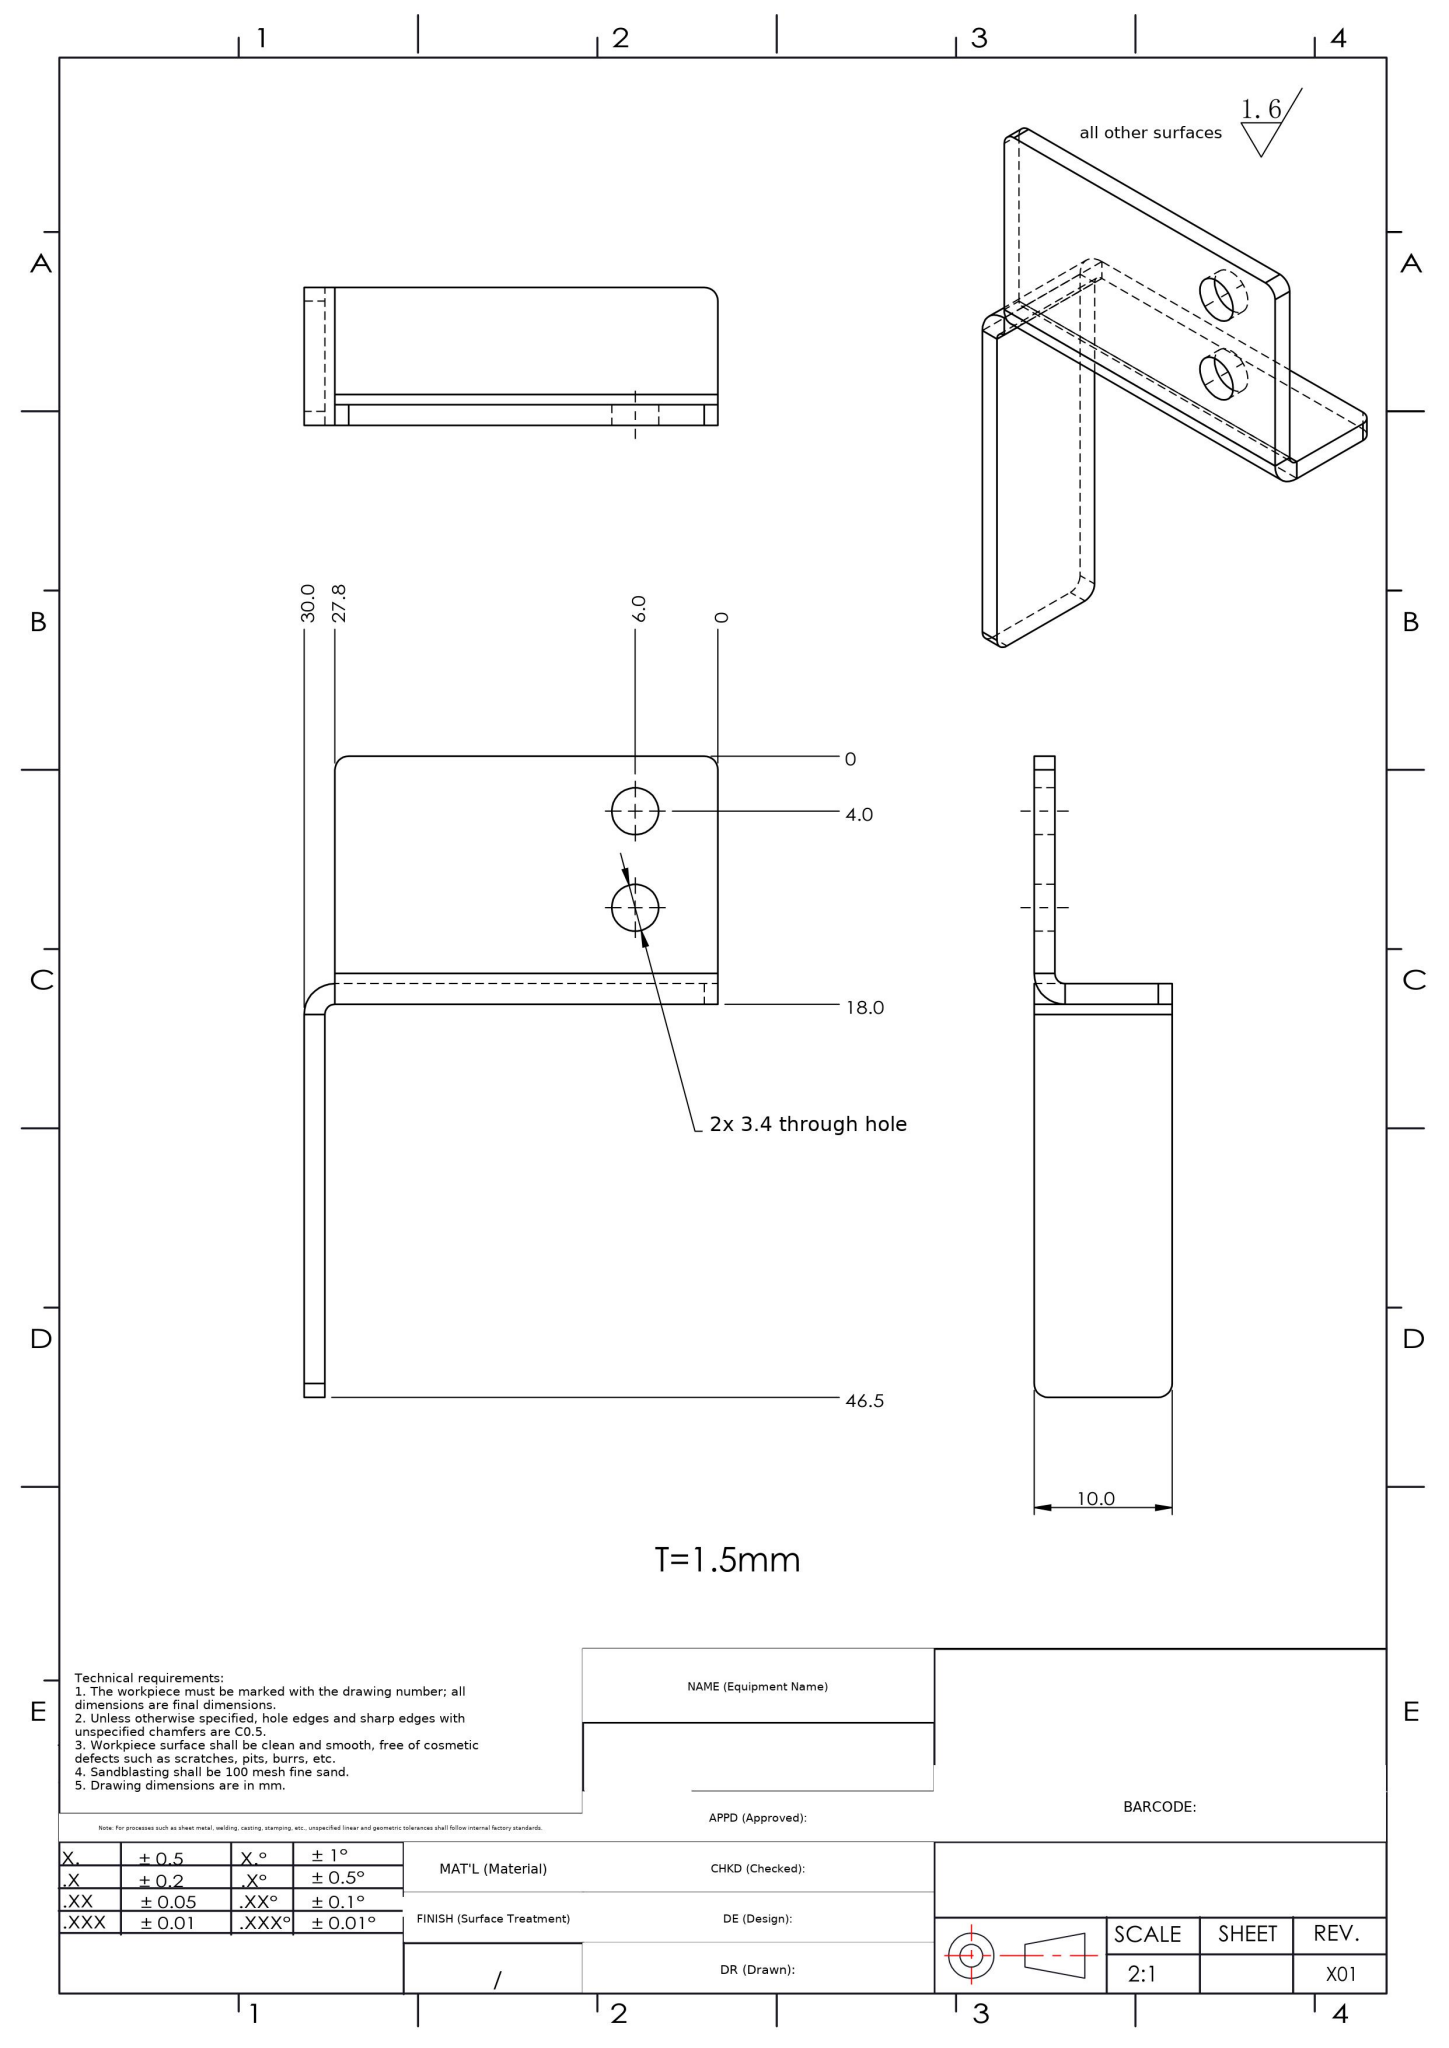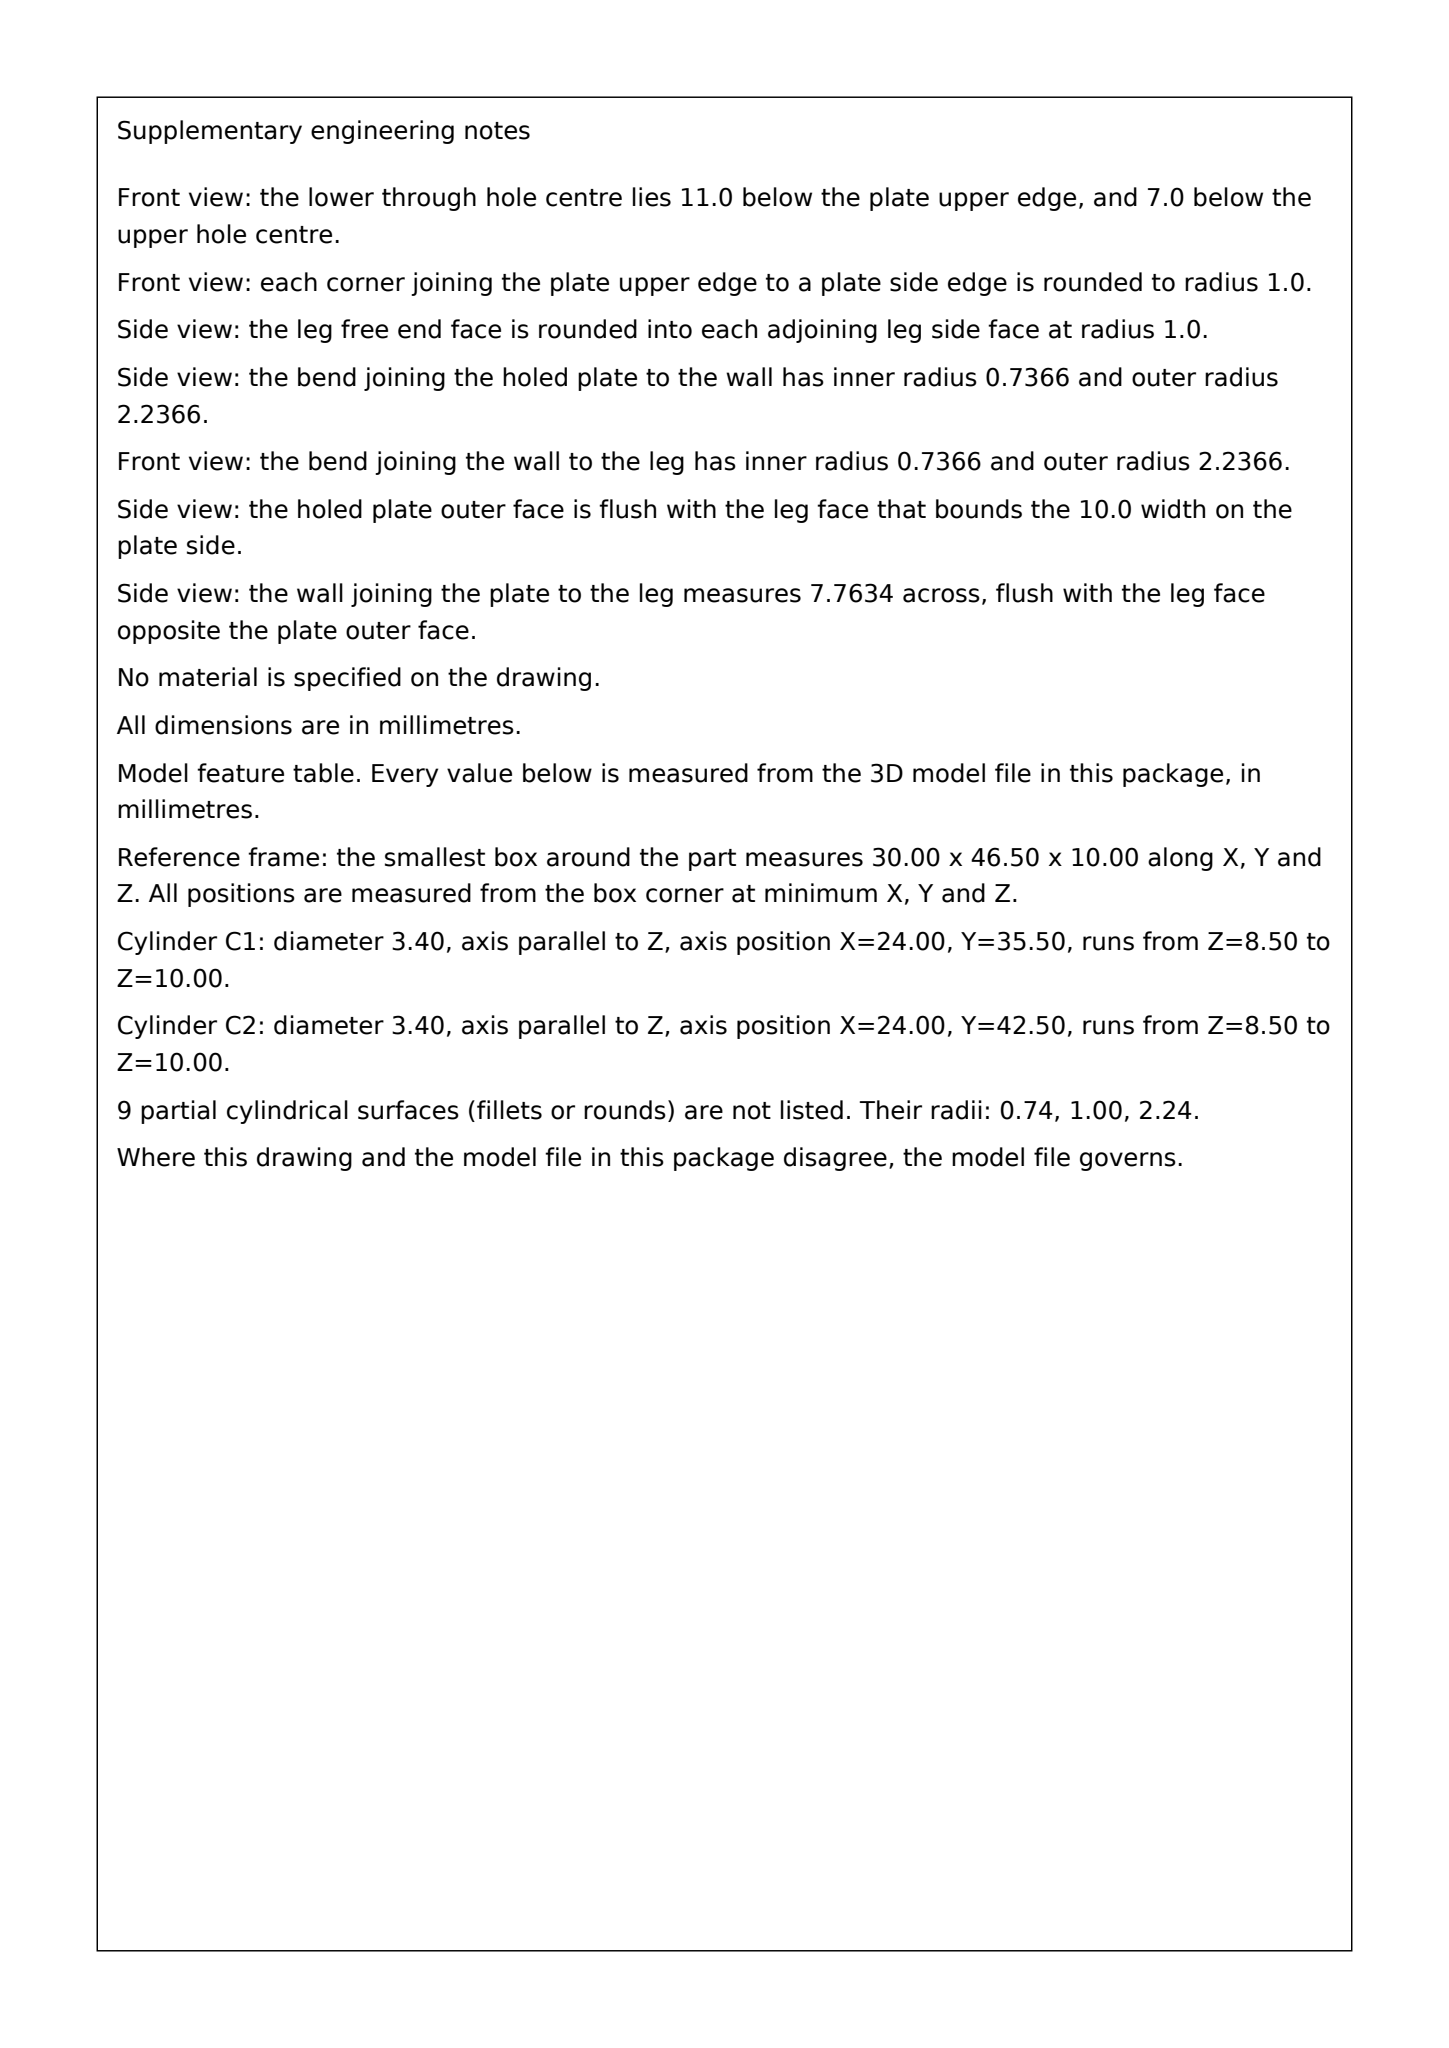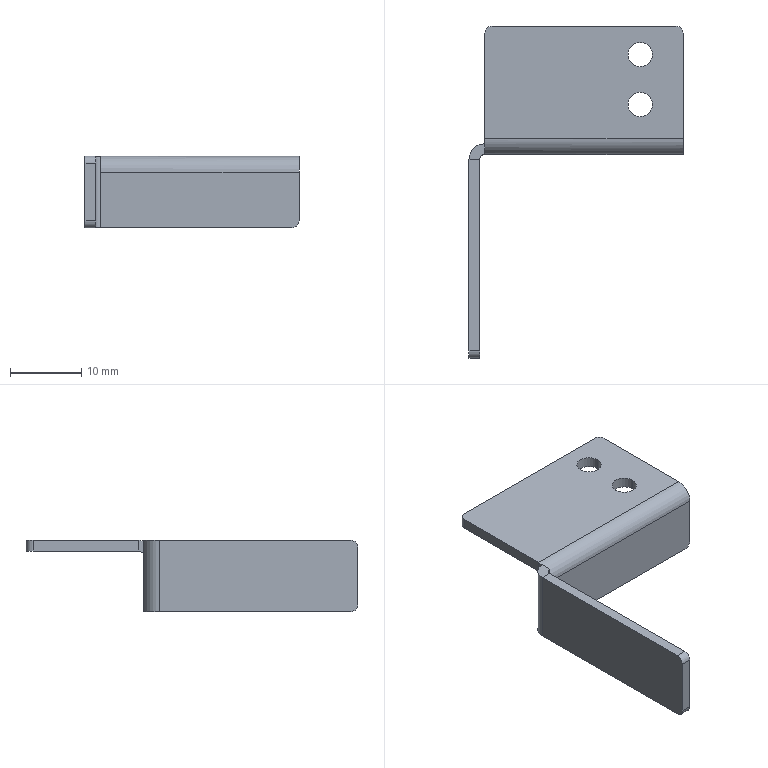Part | SolidWorks | mm | 1 solid | 32 faces | box 30 x 46.5 x 10 mm | volume 1500 mm3 | plane 19 | cylinder 13 | commonest cylinder face diameters 2 x5 3.4 x4 4.473 x2 1.473 x2
Drawing notes:
2X 90° BEND: INSIDE R0.74, OUTSIDE R2.24, T=1.5 | from the solid: Bend cylinders dia 1.473 (R0.736 inner) & dia 4.473 (R2.236 outer), axes x@[30.74,7.76] L27.76 and z@[2.24,27.76] L10.0; thickness 1.5
STEP:
#1=CARTESIAN_POINT('',(25.7,42.5,10.));
#2=VERTEX_POINT('',#1);
#3=CARTESIAN_POINT('',(22.3,42.5,10.));
#4=VERTEX_POINT('',#3);
#5=CARTESIAN_POINT('',(24.,42.5,10.));
#6=DIRECTION('',(0.,0.,-1.));
#7=DIRECTION('',(-1.,0.,0.));
#8=AXIS2_PLACEMENT_3D('',#5,#6,#7);
#9=CIRCLE('',#8,1.7);
#10=EDGE_CURVE('',#2,#4,#9,.T.);
#11=ORIENTED_EDGE('',*,*,#10,.F.);
#12=CARTESIAN_POINT('',(25.7,42.5,8.5));
#13=VERTEX_POINT('',#12);
#14=CARTESIAN_POINT('',(25.7,42.5,8.5));
#15=DIRECTION('',(0.,0.,-1.));
#16=VECTOR('',#15,1000.);
#17=LINE('',#14,#16);
#18=EDGE_CURVE('',#2,#13,#17,.T.);
#19=ORIENTED_EDGE('',*,*,#18,.T.);
#20=CARTESIAN_POINT('',(22.3,42.5,8.5));
#21=VERTEX_POINT('',#20);
#22=CARTESIAN_POINT('',(24.,42.5,8.5));
#23=DIRECTION('',(0.,0.,-1.));
#24=DIRECTION('',(-1.,0.,0.));
#25=AXIS2_PLACEMENT_3D('',#22,#23,#24);
#26=CIRCLE('',#25,1.7);
#27=EDGE_CURVE('',#13,#21,#26,.T.);
#28=ORIENTED_EDGE('',*,*,#27,.T.);
#29=CARTESIAN_POINT('',(22.3,42.5,8.5));
#30=DIRECTION('',(0.,0.,-1.));
#31=VECTOR('',#30,1000.);
#32=LINE('',#29,#31);
#33=EDGE_CURVE('',#4,#21,#32,.T.);
#34=ORIENTED_EDGE('',*,*,#33,.F.);
#35=EDGE_LOOP('',(#11,#19,#28,#34));
#36=FACE_OUTER_BOUND('',#35,.T.);
#37=CARTESIAN_POINT('',(24.,42.5,8.5));
#38=DIRECTION('',(0.,0.,-1.));
#39=DIRECTION('',(-1.,0.,0.));
#40=AXIS2_PLACEMENT_3D('',#37,#38,#39);
#41=CYLINDRICAL_SURFACE('',#40,1.7);
#42=ADVANCED_FACE('',(#36),#41,.F.);
#43=CARTESIAN_POINT('',(25.7,35.5,10.));
#44=VERTEX_POINT('',#43);
#45=CARTESIAN_POINT('',(22.3,35.5,10.));
#46=VERTEX_POINT('',#45);
#47=CARTESIAN_POINT('',(24.,35.5,10.));
#48=DIRECTION('',(0.,0.,-1.));
#49=DIRECTION('',(-1.,0.,0.));
#50=AXIS2_PLACEMENT_3D('',#47,#48,#49);
#51=CIRCLE('',#50,1.7);
#52=EDGE_CURVE('',#44,#46,#51,.T.);
#53=ORIENTED_EDGE('',*,*,#52,.F.);
#54=CARTESIAN_POINT('',(25.7,35.5,8.5));
#55=VERTEX_POINT('',#54);
#56=CARTESIAN_POINT('',(25.7,35.5,8.5));
#57=DIRECTION('',(0.,0.,-1.));
#58=VECTOR('',#57,1000.);
#59=LINE('',#56,#58);
#60=EDGE_CURVE('',#44,#55,#59,.T.);
#61=ORIENTED_EDGE('',*,*,#60,.T.);
#62=CARTESIAN_POINT('',(22.3,35.5,8.5));
#63=VERTEX_POINT('',#62);
#64=CARTESIAN_POINT('',(24.,35.5,8.5));
#65=DIRECTION('',(0.,0.,-1.));
#66=DIRECTION('',(-1.,0.,0.));
#67=AXIS2_PLACEMENT_3D('',#64,#65,#66);
#68=CIRCLE('',#67,1.7);
#69=EDGE_CURVE('',#55,#63,#68,.T.);
#70=ORIENTED_EDGE('',*,*,#69,.T.);
#71=CARTESIAN_POINT('',(22.3,35.5,8.5));
#72=DIRECTION('',(0.,0.,-1.));
#73=VECTOR('',#72,1000.);
#74=LINE('',#71,#73);
#75=EDGE_CURVE('',#46,#63,#74,.T.);
#76=ORIENTED_EDGE('',*,*,#75,.F.);
#77=EDGE_LOOP('',(#53,#61,#70,#76));
#78=FACE_OUTER_BOUND('',#77,.T.);
#79=CARTESIAN_POINT('',(24.,35.5,8.5));
#80=DIRECTION('',(0.,0.,-1.));
#81=DIRECTION('',(-1.,0.,0.));
#82=AXIS2_PLACEMENT_3D('',#79,#80,#81);
#83=CYLINDRICAL_SURFACE('',#82,1.7);
#84=ADVANCED_FACE('',(#78),#83,.F.);
#85=CARTESIAN_POINT('',(2.237,28.5,10.));
#86=VERTEX_POINT('',#85);
#87=CARTESIAN_POINT('',(2.237,28.5,7.763));
#88=VERTEX_POINT('',#87);
#89=CARTESIAN_POINT('',(2.237,28.5,10.));
#90=DIRECTION('',(0.,0.,-1.));
#91=VECTOR('',#90,1000.);
#92=LINE('',#89,#91);
#93=EDGE_CURVE('',#86,#88,#92,.T.);
#94=ORIENTED_EDGE('',*,*,#93,.T.);
#95=CARTESIAN_POINT('',(2.237,30.,9.875));
#96=VERTEX_POINT('',#95);
#97=CARTESIAN_POINT('',(2.237,30.737,7.763));
#98=DIRECTION('',(-1.,0.,0.));
#99=DIRECTION('',(0.,0.,-1.));
#100=AXIS2_PLACEMENT_3D('',#97,#98,#99);
#101=CIRCLE('',#100,2.237);
#102=EDGE_CURVE('',#88,#96,#101,.T.);
#103=ORIENTED_EDGE('',*,*,#102,.T.);
#104=CARTESIAN_POINT('',(2.237,30.,10.));
#105=VERTEX_POINT('',#104);
#106=CARTESIAN_POINT('',(2.237,30.,10.));
#107=DIRECTION('',(0.,0.,-1.));
#108=VECTOR('',#107,1000.);
#109=LINE('',#106,#108);
#110=EDGE_CURVE('',#105,#96,#109,.T.);
#111=ORIENTED_EDGE('',*,*,#110,.F.);
#112=CARTESIAN_POINT('',(2.237,30.,10.));
#113=DIRECTION('',(0.,-1.,0.));
#114=VECTOR('',#113,1000.);
#115=LINE('',#112,#114);
#116=EDGE_CURVE('',#105,#86,#115,.T.);
#117=ORIENTED_EDGE('',*,*,#116,.T.);
#118=EDGE_LOOP('',(#94,#103,#111,#117));
#119=FACE_OUTER_BOUND('',#118,.T.);
#120=CARTESIAN_POINT('',(2.237,30.,7.763));
#121=DIRECTION('',(1.,0.,0.));
#122=DIRECTION('',(0.,0.,-1.));
#123=AXIS2_PLACEMENT_3D('',#120,#121,#122);
#124=PLANE('',#123);
#125=ADVANCED_FACE('',(#119),#124,.T.);
#126=CARTESIAN_POINT('',(2.237,28.5,0.));
#127=VERTEX_POINT('',#126);
#128=CARTESIAN_POINT('',(29.,28.5,0.));
#129=VERTEX_POINT('',#128);
#130=CARTESIAN_POINT('',(0.,28.5,0.));
#131=DIRECTION('',(1.,0.,0.));
#132=VECTOR('',#131,1000.);
#133=LINE('',#130,#132);
#134=EDGE_CURVE('',#127,#129,#133,.T.);
#135=ORIENTED_EDGE('',*,*,#134,.T.);
#136=CARTESIAN_POINT('',(30.,28.5,1.));
#137=VERTEX_POINT('',#136);
#138=CARTESIAN_POINT('',(29.,28.5,1.));
#139=DIRECTION('',(0.,-1.,0.));
#140=DIRECTION('',(0.,0.,1.));
#141=AXIS2_PLACEMENT_3D('',#138,#139,#140);
#142=CIRCLE('',#141,1.);
#143=EDGE_CURVE('',#129,#137,#142,.T.);
#144=ORIENTED_EDGE('',*,*,#143,.T.);
#145=CARTESIAN_POINT('',(30.,28.5,7.763));
#146=VERTEX_POINT('',#145);
#147=CARTESIAN_POINT('',(30.,28.5,10.));
#148=DIRECTION('',(0.,0.,-1.));
#149=VECTOR('',#148,1000.);
#150=LINE('',#147,#149);
#151=EDGE_CURVE('',#146,#137,#150,.T.);
#152=ORIENTED_EDGE('',*,*,#151,.F.);
#153=CARTESIAN_POINT('',(30.,28.5,7.763));
#154=DIRECTION('',(-1.,0.,0.));
#155=VECTOR('',#154,1000.);
#156=LINE('',#153,#155);
#157=EDGE_CURVE('',#146,#88,#156,.T.);
#158=ORIENTED_EDGE('',*,*,#157,.T.);
#159=CARTESIAN_POINT('',(2.237,28.5,10.));
#160=DIRECTION('',(0.,0.,-1.));
#161=VECTOR('',#160,1000.);
#162=LINE('',#159,#161);
#163=EDGE_CURVE('',#88,#127,#162,.T.);
#164=ORIENTED_EDGE('',*,*,#163,.T.);
#165=EDGE_LOOP('',(#135,#144,#152,#158,#164));
#166=FACE_OUTER_BOUND('',#165,.T.);
#167=CARTESIAN_POINT('',(0.,28.5,10.));
#168=DIRECTION('',(0.,1.,0.));
#169=DIRECTION('',(0.,0.,1.));
#170=AXIS2_PLACEMENT_3D('',#167,#168,#169);
#171=PLANE('',#170);
#172=ADVANCED_FACE('',(#166),#171,.F.);
#173=ORIENTED_EDGE('',*,*,#151,.T.);
#174=CARTESIAN_POINT('',(30.,30.,1.));
#175=VERTEX_POINT('',#174);
#176=CARTESIAN_POINT('',(30.,30.,1.));
#177=DIRECTION('',(0.,1.,0.));
#178=VECTOR('',#177,1000.);
#179=LINE('',#176,#178);
#180=EDGE_CURVE('',#137,#175,#179,.T.);
#181=ORIENTED_EDGE('',*,*,#180,.T.);
#182=CARTESIAN_POINT('',(30.,30.,7.763));
#183=VERTEX_POINT('',#182);
#184=CARTESIAN_POINT('',(30.,30.,10.));
#185=DIRECTION('',(0.,0.,-1.));
#186=VECTOR('',#185,1000.);
#187=LINE('',#184,#186);
#188=EDGE_CURVE('',#183,#175,#187,.T.);
#189=ORIENTED_EDGE('',*,*,#188,.F.);
#190=CARTESIAN_POINT('',(30.,30.,7.763));
#191=DIRECTION('',(0.,-1.,0.));
#192=VECTOR('',#191,1000.);
#193=LINE('',#190,#192);
#194=EDGE_CURVE('',#183,#146,#193,.T.);
#195=ORIENTED_EDGE('',*,*,#194,.T.);
#196=EDGE_LOOP('',(#173,#181,#189,#195));
#197=FACE_OUTER_BOUND('',#196,.T.);
#198=CARTESIAN_POINT('',(30.,30.,10.));
#199=DIRECTION('',(1.,0.,0.));
#200=DIRECTION('',(0.,0.,-1.));
#201=AXIS2_PLACEMENT_3D('',#198,#199,#200);
#202=PLANE('',#201);
#203=ADVANCED_FACE('',(#197),#202,.T.);
#204=ORIENTED_EDGE('',*,*,#188,.T.);
#205=CARTESIAN_POINT('',(29.,30.,0.));
#206=VERTEX_POINT('',#205);
#207=CARTESIAN_POINT('',(29.,30.,1.));
#208=DIRECTION('',(0.,1.,0.));
#209=DIRECTION('',(0.,0.,1.));
#210=AXIS2_PLACEMENT_3D('',#207,#208,#209);
#211=CIRCLE('',#210,1.);
#212=EDGE_CURVE('',#175,#206,#211,.T.);
#213=ORIENTED_EDGE('',*,*,#212,.T.);
#214=CARTESIAN_POINT('',(2.237,30.,0.));
#215=VERTEX_POINT('',#214);
#216=CARTESIAN_POINT('',(0.,30.,0.));
#217=DIRECTION('',(1.,0.,0.));
#218=VECTOR('',#217,1000.);
#219=LINE('',#216,#218);
#220=EDGE_CURVE('',#215,#206,#219,.T.);
#221=ORIENTED_EDGE('',*,*,#220,.F.);
#222=CARTESIAN_POINT('',(2.237,30.,7.763));
#223=VERTEX_POINT('',#222);
#224=CARTESIAN_POINT('',(2.237,30.,10.));
#225=DIRECTION('',(0.,0.,-1.));
#226=VECTOR('',#225,1000.);
#227=LINE('',#224,#226);
#228=EDGE_CURVE('',#223,#215,#227,.T.);
#229=ORIENTED_EDGE('',*,*,#228,.F.);
#230=CARTESIAN_POINT('',(30.,30.,7.763));
#231=DIRECTION('',(-1.,0.,0.));
#232=VECTOR('',#231,1000.);
#233=LINE('',#230,#232);
#234=EDGE_CURVE('',#183,#223,#233,.T.);
#235=ORIENTED_EDGE('',*,*,#234,.F.);
#236=EDGE_LOOP('',(#204,#213,#221,#229,#235));
#237=FACE_OUTER_BOUND('',#236,.T.);
#238=CARTESIAN_POINT('',(0.,30.,10.));
#239=DIRECTION('',(0.,1.,0.));
#240=DIRECTION('',(0.,0.,1.));
#241=AXIS2_PLACEMENT_3D('',#238,#239,#240);
#242=PLANE('',#241);
#243=ADVANCED_FACE('',(#237),#242,.T.);
#244=ORIENTED_EDGE('',*,*,#116,.F.);
#245=CARTESIAN_POINT('',(0.,27.763,10.));
#246=VERTEX_POINT('',#245);
#247=CARTESIAN_POINT('',(2.237,27.763,10.));
#248=DIRECTION('',(0.,0.,-1.));
#249=DIRECTION('',(1.,0.,0.));
#250=AXIS2_PLACEMENT_3D('',#247,#248,#249);
#251=CIRCLE('',#250,2.237);
#252=EDGE_CURVE('',#246,#105,#251,.T.);
#253=ORIENTED_EDGE('',*,*,#252,.F.);
#254=CARTESIAN_POINT('',(1.5,27.763,10.));
#255=VERTEX_POINT('',#254);
#256=CARTESIAN_POINT('',(1.5,27.763,10.));
#257=DIRECTION('',(-1.,0.,0.));
#258=VECTOR('',#257,1000.);
#259=LINE('',#256,#258);
#260=EDGE_CURVE('',#255,#246,#259,.T.);
#261=ORIENTED_EDGE('',*,*,#260,.F.);
#262=CARTESIAN_POINT('',(2.237,27.763,10.));
#263=DIRECTION('',(0.,0.,-1.));
#264=DIRECTION('',(1.,0.,0.));
#265=AXIS2_PLACEMENT_3D('',#262,#263,#264);
#266=CIRCLE('',#265,0.7366);
#267=EDGE_CURVE('',#255,#86,#266,.T.);
#268=ORIENTED_EDGE('',*,*,#267,.T.);
#269=EDGE_LOOP('',(#244,#253,#261,#268));
#270=FACE_OUTER_BOUND('',#269,.T.);
#271=CARTESIAN_POINT('',(2.237,30.,10.));
#272=DIRECTION('',(0.,0.,1.));
#273=DIRECTION('',(1.,0.,0.));
#274=AXIS2_PLACEMENT_3D('',#271,#272,#273);
#275=PLANE('',#274);
#276=ADVANCED_FACE('',(#270),#275,.T.);
#277=CARTESIAN_POINT('',(0.,27.763,0.));
#278=VERTEX_POINT('',#277);
#279=CARTESIAN_POINT('',(1.5,27.763,0.));
#280=VERTEX_POINT('',#279);
#281=CARTESIAN_POINT('',(0.,27.763,0.));
#282=DIRECTION('',(1.,0.,0.));
#283=VECTOR('',#282,1000.);
#284=LINE('',#281,#283);
#285=EDGE_CURVE('',#278,#280,#284,.T.);
#286=ORIENTED_EDGE('',*,*,#285,.F.);
#287=CARTESIAN_POINT('',(2.237,27.763,0.));
#288=DIRECTION('',(0.,0.,-1.));
#289=DIRECTION('',(1.,0.,0.));
#290=AXIS2_PLACEMENT_3D('',#287,#288,#289);
#291=CIRCLE('',#290,2.237);
#292=EDGE_CURVE('',#278,#215,#291,.T.);
#293=ORIENTED_EDGE('',*,*,#292,.T.);
#294=CARTESIAN_POINT('',(2.237,28.5,0.));
#295=DIRECTION('',(0.,1.,0.));
#296=VECTOR('',#295,1000.);
#297=LINE('',#294,#296);
#298=EDGE_CURVE('',#127,#215,#297,.T.);
#299=ORIENTED_EDGE('',*,*,#298,.F.);
#300=CARTESIAN_POINT('',(2.237,27.763,0.));
#301=DIRECTION('',(0.,0.,-1.));
#302=DIRECTION('',(1.,0.,0.));
#303=AXIS2_PLACEMENT_3D('',#300,#301,#302);
#304=CIRCLE('',#303,0.7366);
#305=EDGE_CURVE('',#280,#127,#304,.T.);
#306=ORIENTED_EDGE('',*,*,#305,.F.);
#307=EDGE_LOOP('',(#286,#293,#299,#306));
#308=FACE_OUTER_BOUND('',#307,.T.);
#309=CARTESIAN_POINT('',(0.,27.763,0.));
#310=DIRECTION('',(0.,0.,-1.));
#311=DIRECTION('',(-1.,0.,0.));
#312=AXIS2_PLACEMENT_3D('',#309,#310,#311);
#313=PLANE('',#312);
#314=ADVANCED_FACE('',(#308),#313,.T.);
#315=CARTESIAN_POINT('',(1.5,1.,0.));
#316=VERTEX_POINT('',#315);
#317=CARTESIAN_POINT('',(1.5,0.,0.));
#318=DIRECTION('',(0.,1.,0.));
#319=VECTOR('',#318,1000.);
#320=LINE('',#317,#319);
#321=EDGE_CURVE('',#316,#280,#320,.T.);
#322=ORIENTED_EDGE('',*,*,#321,.F.);
#323=CARTESIAN_POINT('',(0.,1.,0.));
#324=VERTEX_POINT('',#323);
#325=CARTESIAN_POINT('',(2.237,1.,0.));
#326=DIRECTION('',(-1.,0.,0.));
#327=VECTOR('',#326,1000.);
#328=LINE('',#325,#327);
#329=EDGE_CURVE('',#316,#324,#328,.T.);
#330=ORIENTED_EDGE('',*,*,#329,.T.);
#331=CARTESIAN_POINT('',(0.,0.,0.));
#332=DIRECTION('',(0.,1.,0.));
#333=VECTOR('',#332,1000.);
#334=LINE('',#331,#333);
#335=EDGE_CURVE('',#324,#278,#334,.T.);
#336=ORIENTED_EDGE('',*,*,#335,.T.);
#337=ORIENTED_EDGE('',*,*,#285,.T.);
#338=EDGE_LOOP('',(#322,#330,#336,#337));
#339=FACE_OUTER_BOUND('',#338,.T.);
#340=CARTESIAN_POINT('',(2.237,28.5,0.));
#341=DIRECTION('',(0.,0.,-1.));
#342=DIRECTION('',(-1.,0.,0.));
#343=AXIS2_PLACEMENT_3D('',#340,#341,#342);
#344=PLANE('',#343);
#345=ADVANCED_FACE('',(#339),#344,.T.);
#346=ORIENTED_EDGE('',*,*,#292,.F.);
#347=CARTESIAN_POINT('',(0.,27.763,10.));
#348=DIRECTION('',(0.,0.,-1.));
#349=VECTOR('',#348,1000.);
#350=LINE('',#347,#349);
#351=EDGE_CURVE('',#246,#278,#350,.T.);
#352=ORIENTED_EDGE('',*,*,#351,.F.);
#353=ORIENTED_EDGE('',*,*,#252,.T.);
#354=ORIENTED_EDGE('',*,*,#110,.T.);
#355=CARTESIAN_POINT('',(2.237,30.,10.));
#356=DIRECTION('',(0.,0.,-1.));
#357=VECTOR('',#356,1000.);
#358=LINE('',#355,#357);
#359=EDGE_CURVE('',#96,#223,#358,.T.);
#360=ORIENTED_EDGE('',*,*,#359,.T.);
#361=ORIENTED_EDGE('',*,*,#228,.T.);
#362=EDGE_LOOP('',(#346,#352,#353,#354,#360,#361));
#363=FACE_OUTER_BOUND('',#362,.T.);
#364=CARTESIAN_POINT('',(2.237,27.763,10.));
#365=DIRECTION('',(0.,0.,-1.));
#366=DIRECTION('',(-1.,0.,0.));
#367=AXIS2_PLACEMENT_3D('',#364,#365,#366);
#368=CYLINDRICAL_SURFACE('',#367,2.237);
#369=ADVANCED_FACE('',(#363),#368,.T.);
#370=ORIENTED_EDGE('',*,*,#335,.F.);
#371=CARTESIAN_POINT('',(0.,0.,1.));
#372=VERTEX_POINT('',#371);
#373=CARTESIAN_POINT('',(0.,1.,1.));
#374=DIRECTION('',(-1.,0.,0.));
#375=DIRECTION('',(0.,0.,1.));
#376=AXIS2_PLACEMENT_3D('',#373,#374,#375);
#377=CIRCLE('',#376,1.);
#378=EDGE_CURVE('',#324,#372,#377,.T.);
#379=ORIENTED_EDGE('',*,*,#378,.T.);
#380=CARTESIAN_POINT('',(0.,0.,9.));
#381=VERTEX_POINT('',#380);
#382=CARTESIAN_POINT('',(0.,0.,10.));
#383=DIRECTION('',(0.,0.,-1.));
#384=VECTOR('',#383,1000.);
#385=LINE('',#382,#384);
#386=EDGE_CURVE('',#381,#372,#385,.T.);
#387=ORIENTED_EDGE('',*,*,#386,.F.);
#388=CARTESIAN_POINT('',(0.,1.,10.));
#389=VERTEX_POINT('',#388);
#390=CARTESIAN_POINT('',(0.,1.,9.));
#391=DIRECTION('',(-1.,0.,0.));
#392=DIRECTION('',(0.,0.,1.));
#393=AXIS2_PLACEMENT_3D('',#390,#391,#392);
#394=CIRCLE('',#393,1.);
#395=EDGE_CURVE('',#381,#389,#394,.T.);
#396=ORIENTED_EDGE('',*,*,#395,.T.);
#397=CARTESIAN_POINT('',(0.,0.,10.));
#398=DIRECTION('',(0.,1.,0.));
#399=VECTOR('',#398,1000.);
#400=LINE('',#397,#399);
#401=EDGE_CURVE('',#389,#246,#400,.T.);
#402=ORIENTED_EDGE('',*,*,#401,.T.);
#403=ORIENTED_EDGE('',*,*,#351,.T.);
#404=EDGE_LOOP('',(#370,#379,#387,#396,#402,#403));
#405=FACE_OUTER_BOUND('',#404,.T.);
#406=CARTESIAN_POINT('',(0.,0.,10.));
#407=DIRECTION('',(-1.,0.,0.));
#408=DIRECTION('',(0.,0.,1.));
#409=AXIS2_PLACEMENT_3D('',#406,#407,#408);
#410=PLANE('',#409);
#411=ADVANCED_FACE('',(#405),#410,.T.);
#412=ORIENTED_EDGE('',*,*,#386,.T.);
#413=CARTESIAN_POINT('',(1.5,0.,1.));
#414=VERTEX_POINT('',#413);
#415=CARTESIAN_POINT('',(1.5,0.,1.));
#416=DIRECTION('',(1.,0.,0.));
#417=VECTOR('',#416,1000.);
#418=LINE('',#415,#417);
#419=EDGE_CURVE('',#372,#414,#418,.T.);
#420=ORIENTED_EDGE('',*,*,#419,.T.);
#421=CARTESIAN_POINT('',(1.5,0.,9.));
#422=VERTEX_POINT('',#421);
#423=CARTESIAN_POINT('',(1.5,0.,10.));
#424=DIRECTION('',(0.,0.,-1.));
#425=VECTOR('',#424,1000.);
#426=LINE('',#423,#425);
#427=EDGE_CURVE('',#422,#414,#426,.T.);
#428=ORIENTED_EDGE('',*,*,#427,.F.);
#429=CARTESIAN_POINT('',(1.5,0.,9.));
#430=DIRECTION('',(-1.,0.,0.));
#431=VECTOR('',#430,1000.);
#432=LINE('',#429,#431);
#433=EDGE_CURVE('',#422,#381,#432,.T.);
#434=ORIENTED_EDGE('',*,*,#433,.T.);
#435=EDGE_LOOP('',(#412,#420,#428,#434));
#436=FACE_OUTER_BOUND('',#435,.T.);
#437=CARTESIAN_POINT('',(1.5,0.,10.));
#438=DIRECTION('',(0.,-1.,0.));
#439=DIRECTION('',(0.,0.,-1.));
#440=AXIS2_PLACEMENT_3D('',#437,#438,#439);
#441=PLANE('',#440);
#442=ADVANCED_FACE('',(#436),#441,.T.);
#443=ORIENTED_EDGE('',*,*,#427,.T.);
#444=CARTESIAN_POINT('',(1.5,1.,1.));
#445=DIRECTION('',(1.,0.,0.));
#446=DIRECTION('',(0.,0.,1.));
#447=AXIS2_PLACEMENT_3D('',#444,#445,#446);
#448=CIRCLE('',#447,1.);
#449=EDGE_CURVE('',#414,#316,#448,.T.);
#450=ORIENTED_EDGE('',*,*,#449,.T.);
#451=ORIENTED_EDGE('',*,*,#321,.T.);
#452=CARTESIAN_POINT('',(1.5,27.763,10.));
#453=DIRECTION('',(0.,0.,-1.));
#454=VECTOR('',#453,1000.);
#455=LINE('',#452,#454);
#456=EDGE_CURVE('',#255,#280,#455,.T.);
#457=ORIENTED_EDGE('',*,*,#456,.F.);
#458=CARTESIAN_POINT('',(1.5,1.,10.));
#459=VERTEX_POINT('',#458);
#460=CARTESIAN_POINT('',(1.5,0.,10.));
#461=DIRECTION('',(0.,1.,0.));
#462=VECTOR('',#461,1000.);
#463=LINE('',#460,#462);
#464=EDGE_CURVE('',#459,#255,#463,.T.);
#465=ORIENTED_EDGE('',*,*,#464,.F.);
#466=CARTESIAN_POINT('',(1.5,1.,9.));
#467=DIRECTION('',(1.,0.,0.));
#468=DIRECTION('',(0.,0.,1.));
#469=AXIS2_PLACEMENT_3D('',#466,#467,#468);
#470=CIRCLE('',#469,1.);
#471=EDGE_CURVE('',#459,#422,#470,.T.);
#472=ORIENTED_EDGE('',*,*,#471,.T.);
#473=EDGE_LOOP('',(#443,#450,#451,#457,#465,#472));
#474=FACE_OUTER_BOUND('',#473,.T.);
#475=CARTESIAN_POINT('',(1.5,0.,10.));
#476=DIRECTION('',(-1.,0.,0.));
#477=DIRECTION('',(0.,0.,1.));
#478=AXIS2_PLACEMENT_3D('',#475,#476,#477);
#479=PLANE('',#478);
#480=ADVANCED_FACE('',(#474),#479,.F.);
#481=ORIENTED_EDGE('',*,*,#305,.T.);
#482=ORIENTED_EDGE('',*,*,#163,.F.);
#483=ORIENTED_EDGE('',*,*,#93,.F.);
#484=ORIENTED_EDGE('',*,*,#267,.F.);
#485=ORIENTED_EDGE('',*,*,#456,.T.);
#486=EDGE_LOOP('',(#481,#482,#483,#484,#485));
#487=FACE_OUTER_BOUND('',#486,.T.);
#488=CARTESIAN_POINT('',(2.237,27.763,10.));
#489=DIRECTION('',(0.,0.,-1.));
#490=DIRECTION('',(-1.,0.,0.));
#491=AXIS2_PLACEMENT_3D('',#488,#489,#490);
#492=CYLINDRICAL_SURFACE('',#491,0.7366);
#493=ADVANCED_FACE('',(#487),#492,.F.);
#494=ORIENTED_EDGE('',*,*,#401,.F.);
#495=CARTESIAN_POINT('',(2.237,1.,10.));
#496=DIRECTION('',(1.,0.,0.));
#497=VECTOR('',#496,1000.);
#498=LINE('',#495,#497);
#499=EDGE_CURVE('',#389,#459,#498,.T.);
#500=ORIENTED_EDGE('',*,*,#499,.T.);
#501=ORIENTED_EDGE('',*,*,#464,.T.);
#502=ORIENTED_EDGE('',*,*,#260,.T.);
#503=EDGE_LOOP('',(#494,#500,#501,#502));
#504=FACE_OUTER_BOUND('',#503,.T.);
#505=CARTESIAN_POINT('',(2.237,27.763,10.));
#506=DIRECTION('',(0.,0.,1.));
#507=DIRECTION('',(1.,0.,0.));
#508=AXIS2_PLACEMENT_3D('',#505,#506,#507);
#509=PLANE('',#508);
#510=ADVANCED_FACE('',(#504),#509,.T.);
#511=ORIENTED_EDGE('',*,*,#220,.T.);
#512=CARTESIAN_POINT('',(29.,28.5,0.));
#513=DIRECTION('',(0.,-1.,0.));
#514=VECTOR('',#513,1000.);
#515=LINE('',#512,#514);
#516=EDGE_CURVE('',#206,#129,#515,.T.);
#517=ORIENTED_EDGE('',*,*,#516,.T.);
#518=ORIENTED_EDGE('',*,*,#134,.F.);
#519=ORIENTED_EDGE('',*,*,#298,.T.);
#520=EDGE_LOOP('',(#511,#517,#518,#519));
#521=FACE_OUTER_BOUND('',#520,.T.);
#522=CARTESIAN_POINT('',(2.237,27.763,0.));
#523=DIRECTION('',(0.,0.,1.));
#524=DIRECTION('',(1.,0.,0.));
#525=AXIS2_PLACEMENT_3D('',#522,#523,#524);
#526=PLANE('',#525);
#527=ADVANCED_FACE('',(#521),#526,.F.);
#528=ORIENTED_EDGE('',*,*,#359,.F.);
#529=CARTESIAN_POINT('',(2.237,30.737,10.));
#530=VERTEX_POINT('',#529);
#531=CARTESIAN_POINT('',(2.237,30.737,7.763));
#532=DIRECTION('',(-1.,0.,0.));
#533=DIRECTION('',(0.,0.,-1.));
#534=AXIS2_PLACEMENT_3D('',#531,#532,#533);
#535=CIRCLE('',#534,2.237);
#536=EDGE_CURVE('',#96,#530,#535,.T.);
#537=ORIENTED_EDGE('',*,*,#536,.T.);
#538=CARTESIAN_POINT('',(2.237,30.737,8.5));
#539=VERTEX_POINT('',#538);
#540=CARTESIAN_POINT('',(2.237,30.737,10.));
#541=DIRECTION('',(0.,0.,1.));
#542=VECTOR('',#541,1000.);
#543=LINE('',#540,#542);
#544=EDGE_CURVE('',#539,#530,#543,.T.);
#545=ORIENTED_EDGE('',*,*,#544,.F.);
#546=CARTESIAN_POINT('',(2.237,30.737,7.763));
#547=DIRECTION('',(-1.,0.,0.));
#548=DIRECTION('',(0.,0.,-1.));
#549=AXIS2_PLACEMENT_3D('',#546,#547,#548);
#550=CIRCLE('',#549,0.7366);
#551=EDGE_CURVE('',#223,#539,#550,.T.);
#552=ORIENTED_EDGE('',*,*,#551,.F.);
#553=EDGE_LOOP('',(#528,#537,#545,#552));
#554=FACE_OUTER_BOUND('',#553,.T.);
#555=CARTESIAN_POINT('',(2.237,30.737,7.763));
#556=DIRECTION('',(-1.,0.,0.));
#557=DIRECTION('',(0.,0.,1.));
#558=AXIS2_PLACEMENT_3D('',#555,#556,#557);
#559=PLANE('',#558);
#560=ADVANCED_FACE('',(#554),#559,.T.);
#561=CARTESIAN_POINT('',(30.,30.737,8.5));
#562=VERTEX_POINT('',#561);
#563=CARTESIAN_POINT('',(30.,30.737,7.763));
#564=DIRECTION('',(1.,0.,0.));
#565=DIRECTION('',(0.,0.,-1.));
#566=AXIS2_PLACEMENT_3D('',#563,#564,#565);
#567=CIRCLE('',#566,0.7366);
#568=EDGE_CURVE('',#562,#183,#567,.T.);
#569=ORIENTED_EDGE('',*,*,#568,.F.);
#570=CARTESIAN_POINT('',(30.,30.737,10.));
#571=VERTEX_POINT('',#570);
#572=CARTESIAN_POINT('',(30.,30.737,8.5));
#573=DIRECTION('',(0.,0.,1.));
#574=VECTOR('',#573,1000.);
#575=LINE('',#572,#574);
#576=EDGE_CURVE('',#562,#571,#575,.T.);
#577=ORIENTED_EDGE('',*,*,#576,.T.);
#578=CARTESIAN_POINT('',(30.,30.737,7.763));
#579=DIRECTION('',(1.,0.,0.));
#580=DIRECTION('',(0.,0.,-1.));
#581=AXIS2_PLACEMENT_3D('',#578,#579,#580);
#582=CIRCLE('',#581,2.237);
#583=EDGE_CURVE('',#571,#146,#582,.T.);
#584=ORIENTED_EDGE('',*,*,#583,.T.);
#585=ORIENTED_EDGE('',*,*,#194,.F.);
#586=EDGE_LOOP('',(#569,#577,#584,#585));
#587=FACE_OUTER_BOUND('',#586,.T.);
#588=CARTESIAN_POINT('',(30.,30.737,7.763));
#589=DIRECTION('',(-1.,0.,0.));
#590=DIRECTION('',(0.,0.,1.));
#591=AXIS2_PLACEMENT_3D('',#588,#589,#590);
#592=PLANE('',#591);
#593=ADVANCED_FACE('',(#587),#592,.F.);
#594=ORIENTED_EDGE('',*,*,#157,.F.);
#595=ORIENTED_EDGE('',*,*,#583,.F.);
#596=CARTESIAN_POINT('',(2.237,30.737,10.));
#597=DIRECTION('',(-1.,0.,0.));
#598=VECTOR('',#597,1000.);
#599=LINE('',#596,#598);
#600=EDGE_CURVE('',#571,#530,#599,.T.);
#601=ORIENTED_EDGE('',*,*,#600,.T.);
#602=ORIENTED_EDGE('',*,*,#536,.F.);
#603=ORIENTED_EDGE('',*,*,#102,.F.);
#604=EDGE_LOOP('',(#594,#595,#601,#602,#603));
#605=FACE_OUTER_BOUND('',#604,.T.);
#606=CARTESIAN_POINT('',(30.,30.737,7.763));
#607=DIRECTION('',(1.,0.,0.));
#608=DIRECTION('',(0.,0.,1.));
#609=AXIS2_PLACEMENT_3D('',#606,#607,#608);
#610=CYLINDRICAL_SURFACE('',#609,2.237);
#611=ADVANCED_FACE('',(#605),#610,.T.);
#612=ORIENTED_EDGE('',*,*,#234,.T.);
#613=ORIENTED_EDGE('',*,*,#551,.T.);
#614=CARTESIAN_POINT('',(2.237,30.737,8.5));
#615=DIRECTION('',(1.,0.,0.));
#616=VECTOR('',#615,1000.);
#617=LINE('',#614,#616);
#618=EDGE_CURVE('',#539,#562,#617,.T.);
#619=ORIENTED_EDGE('',*,*,#618,.T.);
#620=ORIENTED_EDGE('',*,*,#568,.T.);
#621=EDGE_LOOP('',(#612,#613,#619,#620));
#622=FACE_OUTER_BOUND('',#621,.T.);
#623=CARTESIAN_POINT('',(30.,30.737,7.763));
#624=DIRECTION('',(1.,0.,0.));
#625=DIRECTION('',(0.,0.,1.));
#626=AXIS2_PLACEMENT_3D('',#623,#624,#625);
#627=CYLINDRICAL_SURFACE('',#626,0.7366);
#628=ADVANCED_FACE('',(#622),#627,.F.);
#629=CARTESIAN_POINT('',(2.237,45.5,10.));
#630=VERTEX_POINT('',#629);
#631=CARTESIAN_POINT('',(2.237,0.,10.));
#632=DIRECTION('',(0.,-1.,0.));
#633=VECTOR('',#632,1000.);
#634=LINE('',#631,#633);
#635=EDGE_CURVE('',#630,#530,#634,.T.);
#636=ORIENTED_EDGE('',*,*,#635,.F.);
#637=CARTESIAN_POINT('',(2.237,45.5,8.5));
#638=VERTEX_POINT('',#637);
#639=CARTESIAN_POINT('',(2.237,45.5,10.));
#640=DIRECTION('',(0.,0.,-1.));
#641=VECTOR('',#640,1000.);
#642=LINE('',#639,#641);
#643=EDGE_CURVE('',#630,#638,#642,.T.);
#644=ORIENTED_EDGE('',*,*,#643,.T.);
#645=CARTESIAN_POINT('',(2.237,30.,8.5));
#646=DIRECTION('',(0.,-1.,0.));
#647=VECTOR('',#646,1000.);
#648=LINE('',#645,#647);
#649=EDGE_CURVE('',#638,#539,#648,.T.);
#650=ORIENTED_EDGE('',*,*,#649,.T.);
#651=ORIENTED_EDGE('',*,*,#544,.T.);
#652=EDGE_LOOP('',(#636,#644,#650,#651));
#653=FACE_OUTER_BOUND('',#652,.T.);
#654=CARTESIAN_POINT('',(2.237,30.,10.));
#655=DIRECTION('',(1.,0.,0.));
#656=DIRECTION('',(0.,0.,-1.));
#657=AXIS2_PLACEMENT_3D('',#654,#655,#656);
#658=PLANE('',#657);
#659=ADVANCED_FACE('',(#653),#658,.F.);
#660=CARTESIAN_POINT('',(30.,45.5,8.5));
#661=VERTEX_POINT('',#660);
#662=CARTESIAN_POINT('',(30.,46.5,8.5));
#663=DIRECTION('',(-0.,1.,0.));
#664=VECTOR('',#663,1000.);
#665=LINE('',#662,#664);
#666=EDGE_CURVE('',#562,#661,#665,.T.);
#667=ORIENTED_EDGE('',*,*,#666,.T.);
#668=CARTESIAN_POINT('',(30.,45.5,10.));
#669=VERTEX_POINT('',#668);
#670=CARTESIAN_POINT('',(30.,45.5,10.));
#671=DIRECTION('',(0.,0.,1.));
#672=VECTOR('',#671,1000.);
#673=LINE('',#670,#672);
#674=EDGE_CURVE('',#661,#669,#673,.T.);
#675=ORIENTED_EDGE('',*,*,#674,.T.);
#676=CARTESIAN_POINT('',(30.,0.,10.));
#677=DIRECTION('',(-0.,1.,0.));
#678=VECTOR('',#677,1000.);
#679=LINE('',#676,#678);
#680=EDGE_CURVE('',#571,#669,#679,.T.);
#681=ORIENTED_EDGE('',*,*,#680,.F.);
#682=ORIENTED_EDGE('',*,*,#576,.F.);
#683=EDGE_LOOP('',(#667,#675,#681,#682));
#684=FACE_OUTER_BOUND('',#683,.T.);
#685=CARTESIAN_POINT('',(30.,46.5,10.));
#686=DIRECTION('',(-1.,-0.,0.));
#687=DIRECTION('',(0.,-1.,0.));
#688=AXIS2_PLACEMENT_3D('',#685,#686,#687);
#689=PLANE('',#688);
#690=ADVANCED_FACE('',(#684),#689,.F.);
#691=CARTESIAN_POINT('',(24.,42.5,10.));
#692=DIRECTION('',(0.,0.,-1.));
#693=DIRECTION('',(-1.,0.,0.));
#694=AXIS2_PLACEMENT_3D('',#691,#692,#693);
#695=CIRCLE('',#694,1.7);
#696=EDGE_CURVE('',#4,#2,#695,.T.);
#697=ORIENTED_EDGE('',*,*,#696,.T.);
#698=ORIENTED_EDGE('',*,*,#10,.T.);
#699=EDGE_LOOP('',(#697,#698));
#700=FACE_BOUND('',#699,.T.);
#701=CARTESIAN_POINT('',(24.,35.5,10.));
#702=DIRECTION('',(0.,0.,-1.));
#703=DIRECTION('',(-1.,0.,0.));
#704=AXIS2_PLACEMENT_3D('',#701,#702,#703);
#705=CIRCLE('',#704,1.7);
#706=EDGE_CURVE('',#46,#44,#705,.T.);
#707=ORIENTED_EDGE('',*,*,#706,.T.);
#708=ORIENTED_EDGE('',*,*,#52,.T.);
#709=EDGE_LOOP('',(#707,#708));
#710=FACE_BOUND('',#709,.T.);
#711=CARTESIAN_POINT('',(29.,46.5,10.));
#712=VERTEX_POINT('',#711);
#713=CARTESIAN_POINT('',(3.237,46.5,10.));
#714=VERTEX_POINT('',#713);
#715=CARTESIAN_POINT('',(0.,46.5,10.));
#716=DIRECTION('',(-1.,0.,0.));
#717=VECTOR('',#716,1000.);
#718=LINE('',#715,#717);
#719=EDGE_CURVE('',#712,#714,#718,.T.);
#720=ORIENTED_EDGE('',*,*,#719,.T.);
#721=CARTESIAN_POINT('',(3.237,45.5,10.));
#722=DIRECTION('',(0.,0.,1.));
#723=DIRECTION('',(-1.,0.,0.));
#724=AXIS2_PLACEMENT_3D('',#721,#722,#723);
#725=CIRCLE('',#724,1.);
#726=EDGE_CURVE('',#714,#630,#725,.T.);
#727=ORIENTED_EDGE('',*,*,#726,.T.);
#728=ORIENTED_EDGE('',*,*,#635,.T.);
#729=ORIENTED_EDGE('',*,*,#600,.F.);
#730=ORIENTED_EDGE('',*,*,#680,.T.);
#731=CARTESIAN_POINT('',(29.,45.5,10.));
#732=DIRECTION('',(0.,0.,1.));
#733=DIRECTION('',(-1.,0.,0.));
#734=AXIS2_PLACEMENT_3D('',#731,#732,#733);
#735=CIRCLE('',#734,1.);
#736=EDGE_CURVE('',#669,#712,#735,.T.);
#737=ORIENTED_EDGE('',*,*,#736,.T.);
#738=EDGE_LOOP('',(#720,#727,#728,#729,#730,#737));
#739=FACE_OUTER_BOUND('',#738,.T.);
#740=CARTESIAN_POINT('',(0.,0.,10.));
#741=DIRECTION('',(0.,0.,-1.));
#742=DIRECTION('',(-1.,0.,0.));
#743=AXIS2_PLACEMENT_3D('',#740,#741,#742);
#744=PLANE('',#743);
#745=ADVANCED_FACE('',(#700,#710,#739),#744,.F.);
#746=CARTESIAN_POINT('',(24.,42.5,8.5));
#747=DIRECTION('',(0.,0.,-1.));
#748=DIRECTION('',(-1.,0.,0.));
#749=AXIS2_PLACEMENT_3D('',#746,#747,#748);
#750=CIRCLE('',#749,1.7);
#751=EDGE_CURVE('',#21,#13,#750,.T.);
#752=ORIENTED_EDGE('',*,*,#751,.F.);
#753=ORIENTED_EDGE('',*,*,#27,.F.);
#754=EDGE_LOOP('',(#752,#753));
#755=FACE_BOUND('',#754,.T.);
#756=CARTESIAN_POINT('',(24.,35.5,8.5));
#757=DIRECTION('',(0.,0.,-1.));
#758=DIRECTION('',(-1.,0.,0.));
#759=AXIS2_PLACEMENT_3D('',#756,#757,#758);
#760=CIRCLE('',#759,1.7);
#761=EDGE_CURVE('',#63,#55,#760,.T.);
#762=ORIENTED_EDGE('',*,*,#761,.F.);
#763=ORIENTED_EDGE('',*,*,#69,.F.);
#764=EDGE_LOOP('',(#762,#763));
#765=FACE_BOUND('',#764,.T.);
#766=ORIENTED_EDGE('',*,*,#649,.F.);
#767=CARTESIAN_POINT('',(3.237,46.5,8.5));
#768=VERTEX_POINT('',#767);
#769=CARTESIAN_POINT('',(3.237,45.5,8.5));
#770=DIRECTION('',(0.,0.,-1.));
#771=DIRECTION('',(-1.,0.,0.));
#772=AXIS2_PLACEMENT_3D('',#769,#770,#771);
#773=CIRCLE('',#772,1.);
#774=EDGE_CURVE('',#638,#768,#773,.T.);
#775=ORIENTED_EDGE('',*,*,#774,.T.);
#776=CARTESIAN_POINT('',(29.,46.5,8.5));
#777=VERTEX_POINT('',#776);
#778=CARTESIAN_POINT('',(2.237,46.5,8.5));
#779=DIRECTION('',(-1.,0.,0.));
#780=VECTOR('',#779,1000.);
#781=LINE('',#778,#780);
#782=EDGE_CURVE('',#777,#768,#781,.T.);
#783=ORIENTED_EDGE('',*,*,#782,.F.);
#784=CARTESIAN_POINT('',(29.,45.5,8.5));
#785=DIRECTION('',(0.,0.,-1.));
#786=DIRECTION('',(-1.,0.,0.));
#787=AXIS2_PLACEMENT_3D('',#784,#785,#786);
#788=CIRCLE('',#787,1.);
#789=EDGE_CURVE('',#777,#661,#788,.T.);
#790=ORIENTED_EDGE('',*,*,#789,.T.);
#791=ORIENTED_EDGE('',*,*,#666,.F.);
#792=ORIENTED_EDGE('',*,*,#618,.F.);
#793=EDGE_LOOP('',(#766,#775,#783,#790,#791,#792));
#794=FACE_OUTER_BOUND('',#793,.T.);
#795=CARTESIAN_POINT('',(0.,0.,8.5));
#796=DIRECTION('',(0.,0.,-1.));
#797=DIRECTION('',(-1.,0.,0.));
#798=AXIS2_PLACEMENT_3D('',#795,#796,#797);
#799=PLANE('',#798);
#800=ADVANCED_FACE('',(#755,#765,#794),#799,.T.);
#801=ORIENTED_EDGE('',*,*,#782,.T.);
#802=CARTESIAN_POINT('',(3.237,46.5,10.));
#803=DIRECTION('',(0.,0.,1.));
#804=VECTOR('',#803,1000.);
#805=LINE('',#802,#804);
#806=EDGE_CURVE('',#768,#714,#805,.T.);
#807=ORIENTED_EDGE('',*,*,#806,.T.);
#808=ORIENTED_EDGE('',*,*,#719,.F.);
#809=CARTESIAN_POINT('',(29.,46.5,10.));
#810=DIRECTION('',(0.,0.,-1.));
#811=VECTOR('',#810,1000.);
#812=LINE('',#809,#811);
#813=EDGE_CURVE('',#712,#777,#812,.T.);
#814=ORIENTED_EDGE('',*,*,#813,.T.);
#815=EDGE_LOOP('',(#801,#807,#808,#814));
#816=FACE_OUTER_BOUND('',#815,.T.);
#817=CARTESIAN_POINT('',(2.237,46.5,10.));
#818=DIRECTION('',(0.,-1.,0.));
#819=DIRECTION('',(0.,0.,-1.));
#820=AXIS2_PLACEMENT_3D('',#817,#818,#819);
#821=PLANE('',#820);
#822=ADVANCED_FACE('',(#816),#821,.F.);
#823=ORIENTED_EDGE('',*,*,#212,.F.);
#824=ORIENTED_EDGE('',*,*,#180,.F.);
#825=ORIENTED_EDGE('',*,*,#143,.F.);
#826=ORIENTED_EDGE('',*,*,#516,.F.);
#827=EDGE_LOOP('',(#823,#824,#825,#826));
#828=FACE_OUTER_BOUND('',#827,.T.);
#829=CARTESIAN_POINT('',(29.,27.763,1.));
#830=DIRECTION('',(0.,1.,0.));
#831=DIRECTION('',(0.,0.,1.));
#832=AXIS2_PLACEMENT_3D('',#829,#830,#831);
#833=CYLINDRICAL_SURFACE('',#832,1.);
#834=ADVANCED_FACE('',(#828),#833,.T.);
#835=ORIENTED_EDGE('',*,*,#726,.F.);
#836=ORIENTED_EDGE('',*,*,#806,.F.);
#837=ORIENTED_EDGE('',*,*,#774,.F.);
#838=ORIENTED_EDGE('',*,*,#643,.F.);
#839=EDGE_LOOP('',(#835,#836,#837,#838));
#840=FACE_OUTER_BOUND('',#839,.T.);
#841=CARTESIAN_POINT('',(3.237,45.5,10.));
#842=DIRECTION('',(0.,0.,-1.));
#843=DIRECTION('',(-1.,0.,0.));
#844=AXIS2_PLACEMENT_3D('',#841,#842,#843);
#845=CYLINDRICAL_SURFACE('',#844,1.);
#846=ADVANCED_FACE('',(#840),#845,.T.);
#847=ORIENTED_EDGE('',*,*,#736,.F.);
#848=ORIENTED_EDGE('',*,*,#674,.F.);
#849=ORIENTED_EDGE('',*,*,#789,.F.);
#850=ORIENTED_EDGE('',*,*,#813,.F.);
#851=EDGE_LOOP('',(#847,#848,#849,#850));
#852=FACE_OUTER_BOUND('',#851,.T.);
#853=CARTESIAN_POINT('',(29.,45.5,10.));
#854=DIRECTION('',(0.,0.,-1.));
#855=DIRECTION('',(-1.,0.,0.));
#856=AXIS2_PLACEMENT_3D('',#853,#854,#855);
#857=CYLINDRICAL_SURFACE('',#856,1.);
#858=ADVANCED_FACE('',(#852),#857,.T.);
#859=ORIENTED_EDGE('',*,*,#449,.F.);
#860=ORIENTED_EDGE('',*,*,#419,.F.);
#861=ORIENTED_EDGE('',*,*,#378,.F.);
#862=ORIENTED_EDGE('',*,*,#329,.F.);
#863=EDGE_LOOP('',(#859,#860,#861,#862));
#864=FACE_OUTER_BOUND('',#863,.T.);
#865=CARTESIAN_POINT('',(2.237,1.,1.));
#866=DIRECTION('',(-1.,0.,0.));
#867=DIRECTION('',(0.,0.,1.));
#868=AXIS2_PLACEMENT_3D('',#865,#866,#867);
#869=CYLINDRICAL_SURFACE('',#868,1.);
#870=ADVANCED_FACE('',(#864),#869,.T.);
#871=ORIENTED_EDGE('',*,*,#471,.F.);
#872=ORIENTED_EDGE('',*,*,#499,.F.);
#873=ORIENTED_EDGE('',*,*,#395,.F.);
#874=ORIENTED_EDGE('',*,*,#433,.F.);
#875=EDGE_LOOP('',(#871,#872,#873,#874));
#876=FACE_OUTER_BOUND('',#875,.T.);
#877=CARTESIAN_POINT('',(1.5,1.,9.));
#878=DIRECTION('',(-1.,0.,0.));
#879=DIRECTION('',(0.,0.,1.));
#880=AXIS2_PLACEMENT_3D('',#877,#878,#879);
#881=CYLINDRICAL_SURFACE('',#880,1.);
#882=ADVANCED_FACE('',(#876),#881,.T.);
#883=ORIENTED_EDGE('',*,*,#60,.F.);
#884=ORIENTED_EDGE('',*,*,#706,.F.);
#885=ORIENTED_EDGE('',*,*,#75,.T.);
#886=ORIENTED_EDGE('',*,*,#761,.T.);
#887=EDGE_LOOP('',(#883,#884,#885,#886));
#888=FACE_OUTER_BOUND('',#887,.T.);
#889=CARTESIAN_POINT('',(24.,35.5,8.5));
#890=DIRECTION('',(0.,0.,-1.));
#891=DIRECTION('',(-1.,0.,0.));
#892=AXIS2_PLACEMENT_3D('',#889,#890,#891);
#893=CYLINDRICAL_SURFACE('',#892,1.7);
#894=ADVANCED_FACE('',(#888),#893,.F.);
#895=ORIENTED_EDGE('',*,*,#18,.F.);
#896=ORIENTED_EDGE('',*,*,#696,.F.);
#897=ORIENTED_EDGE('',*,*,#33,.T.);
#898=ORIENTED_EDGE('',*,*,#751,.T.);
#899=EDGE_LOOP('',(#895,#896,#897,#898));
#900=FACE_OUTER_BOUND('',#899,.T.);
#901=CARTESIAN_POINT('',(24.,42.5,8.5));
#902=DIRECTION('',(0.,0.,-1.));
#903=DIRECTION('',(-1.,0.,0.));
#904=AXIS2_PLACEMENT_3D('',#901,#902,#903);
#905=CYLINDRICAL_SURFACE('',#904,1.7);
#906=ADVANCED_FACE('',(#900),#905,.F.);
#907=CLOSED_SHELL('',(#42,#84,#125,#172,#203,#243,#276,#314,#345,#369,#411,#442,#480,#493,#510,#527,#560,#593,#611,#628,#659,#690,#745,#800,#822,#834,#846,#858,#870,#882,#894,#906));
#908=MANIFOLD_SOLID_BREP('',#907);
#909=CARTESIAN_POINT('',(0.,0.,0.));
#910=DIRECTION('',(0.,0.,1.));
#911=DIRECTION('',(1.,0.,0.));
#912=AXIS2_PLACEMENT_3D('',#909,#910,#911);
#913=(LENGTH_UNIT()NAMED_UNIT(*)SI_UNIT(.MILLI.,.METRE.));
#914=UNCERTAINTY_MEASURE_WITH_UNIT(LENGTH_MEASURE(0.00001),#913,'','');
#915=(NAMED_UNIT(*)PLANE_ANGLE_UNIT()SI_UNIT($,.RADIAN.));
#916=(NAMED_UNIT(*)SI_UNIT($,.STERADIAN.)SOLID_ANGLE_UNIT());
#917=(GEOMETRIC_REPRESENTATION_CONTEXT(3)GLOBAL_UNCERTAINTY_ASSIGNED_CONTEXT((#914))GLOBAL_UNIT_ASSIGNED_CONTEXT((#913,#915,#916))REPRESENTATION_CONTEXT('',''));
#918=ADVANCED_BREP_SHAPE_REPRESENTATION('',(#908,#912),#917);